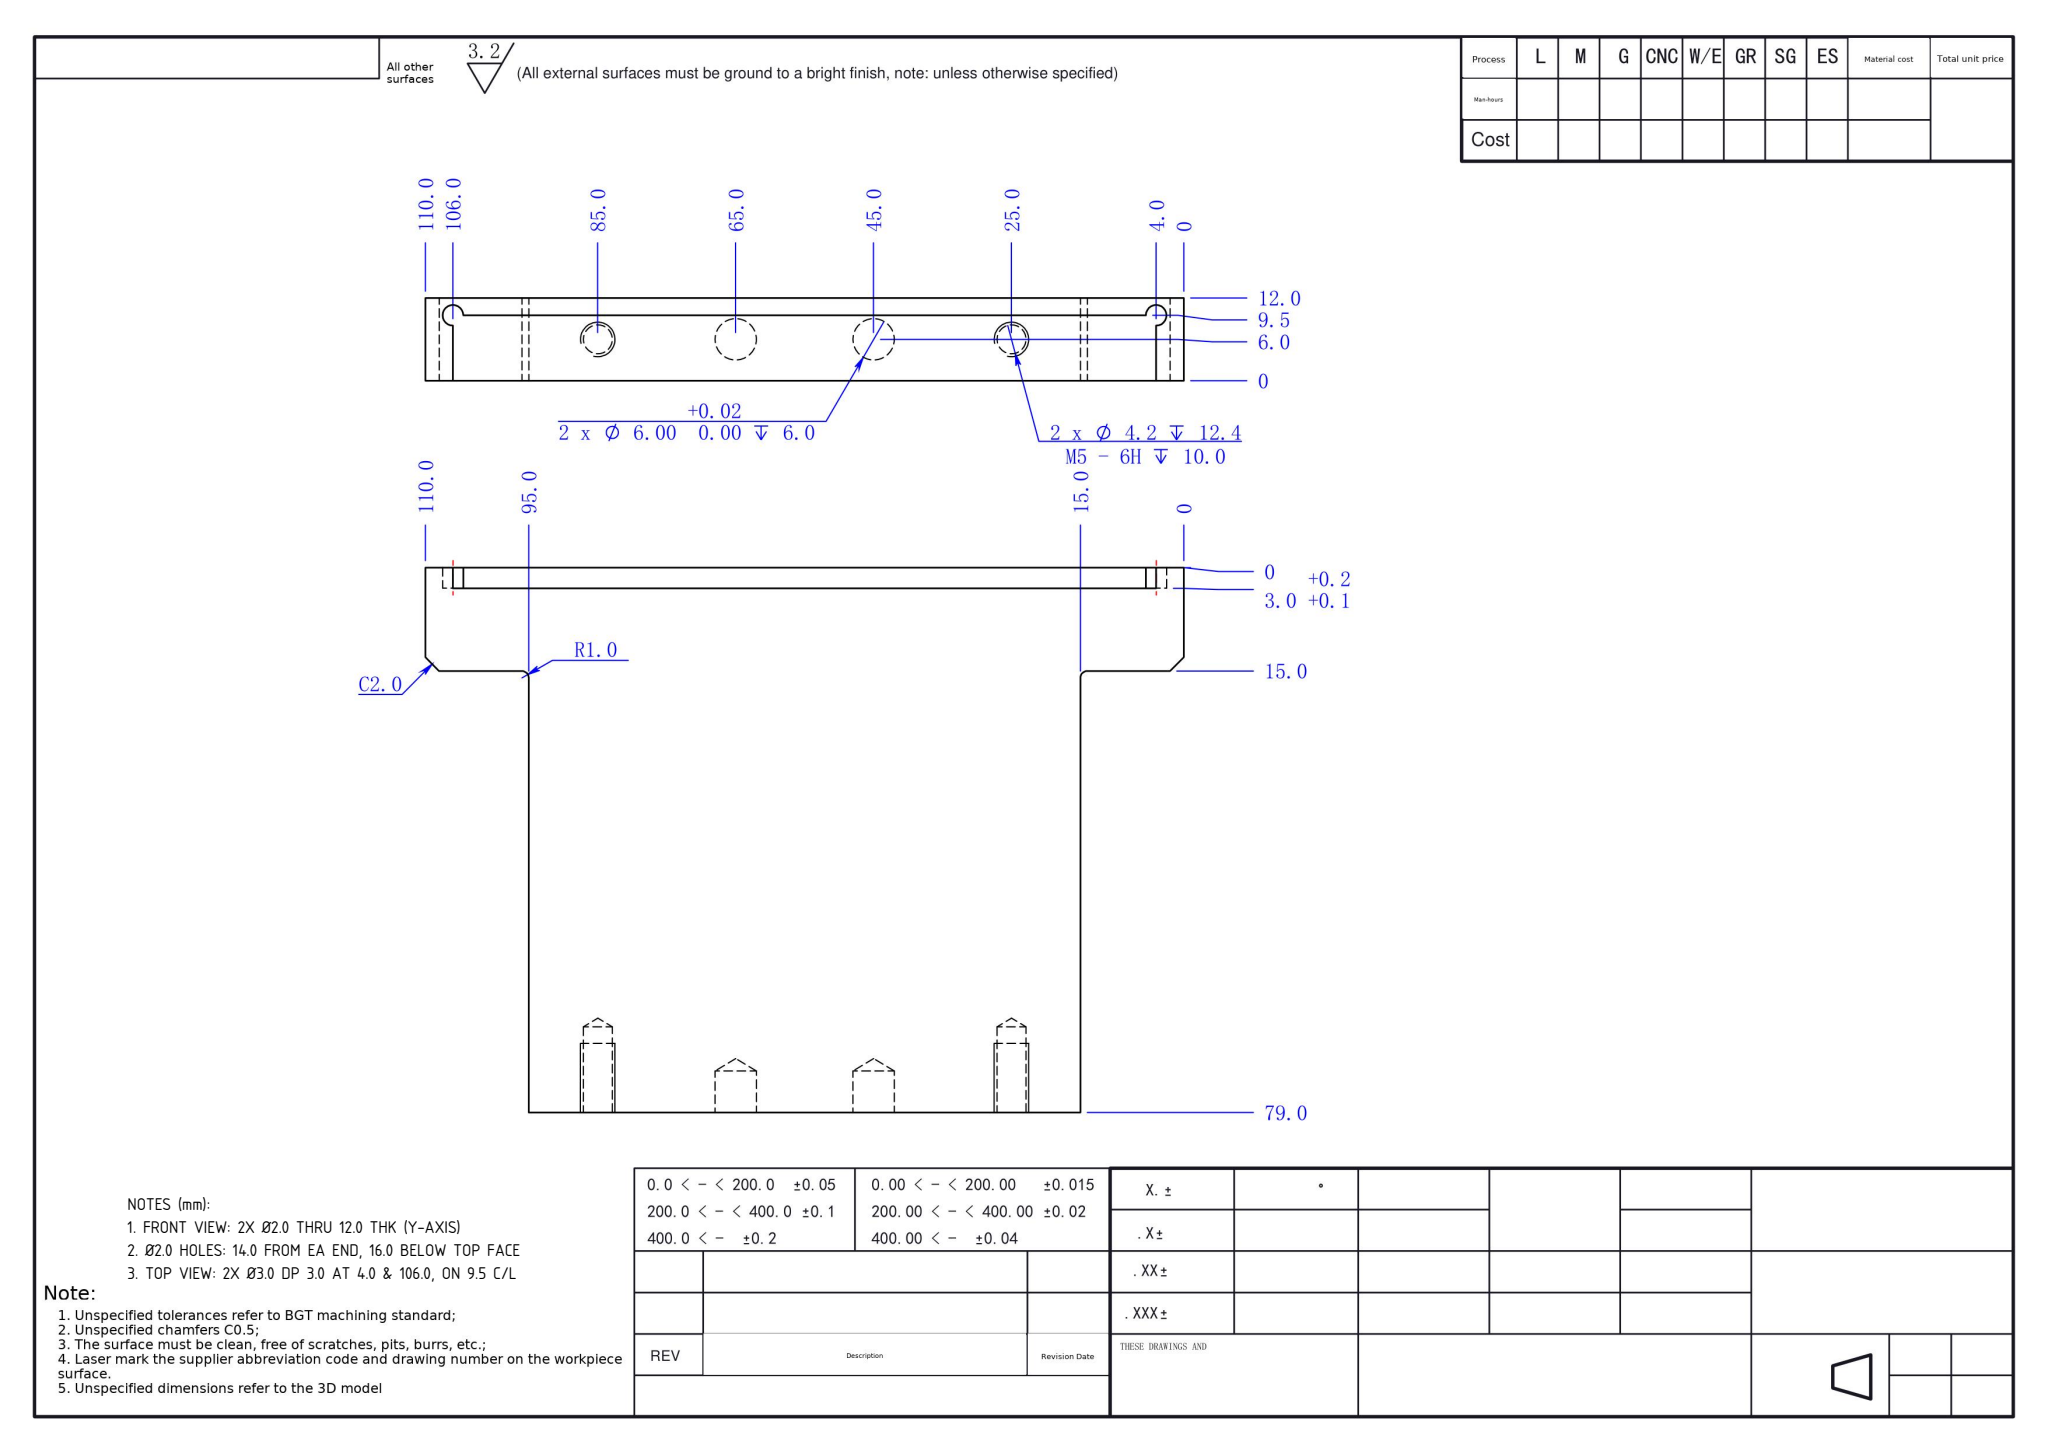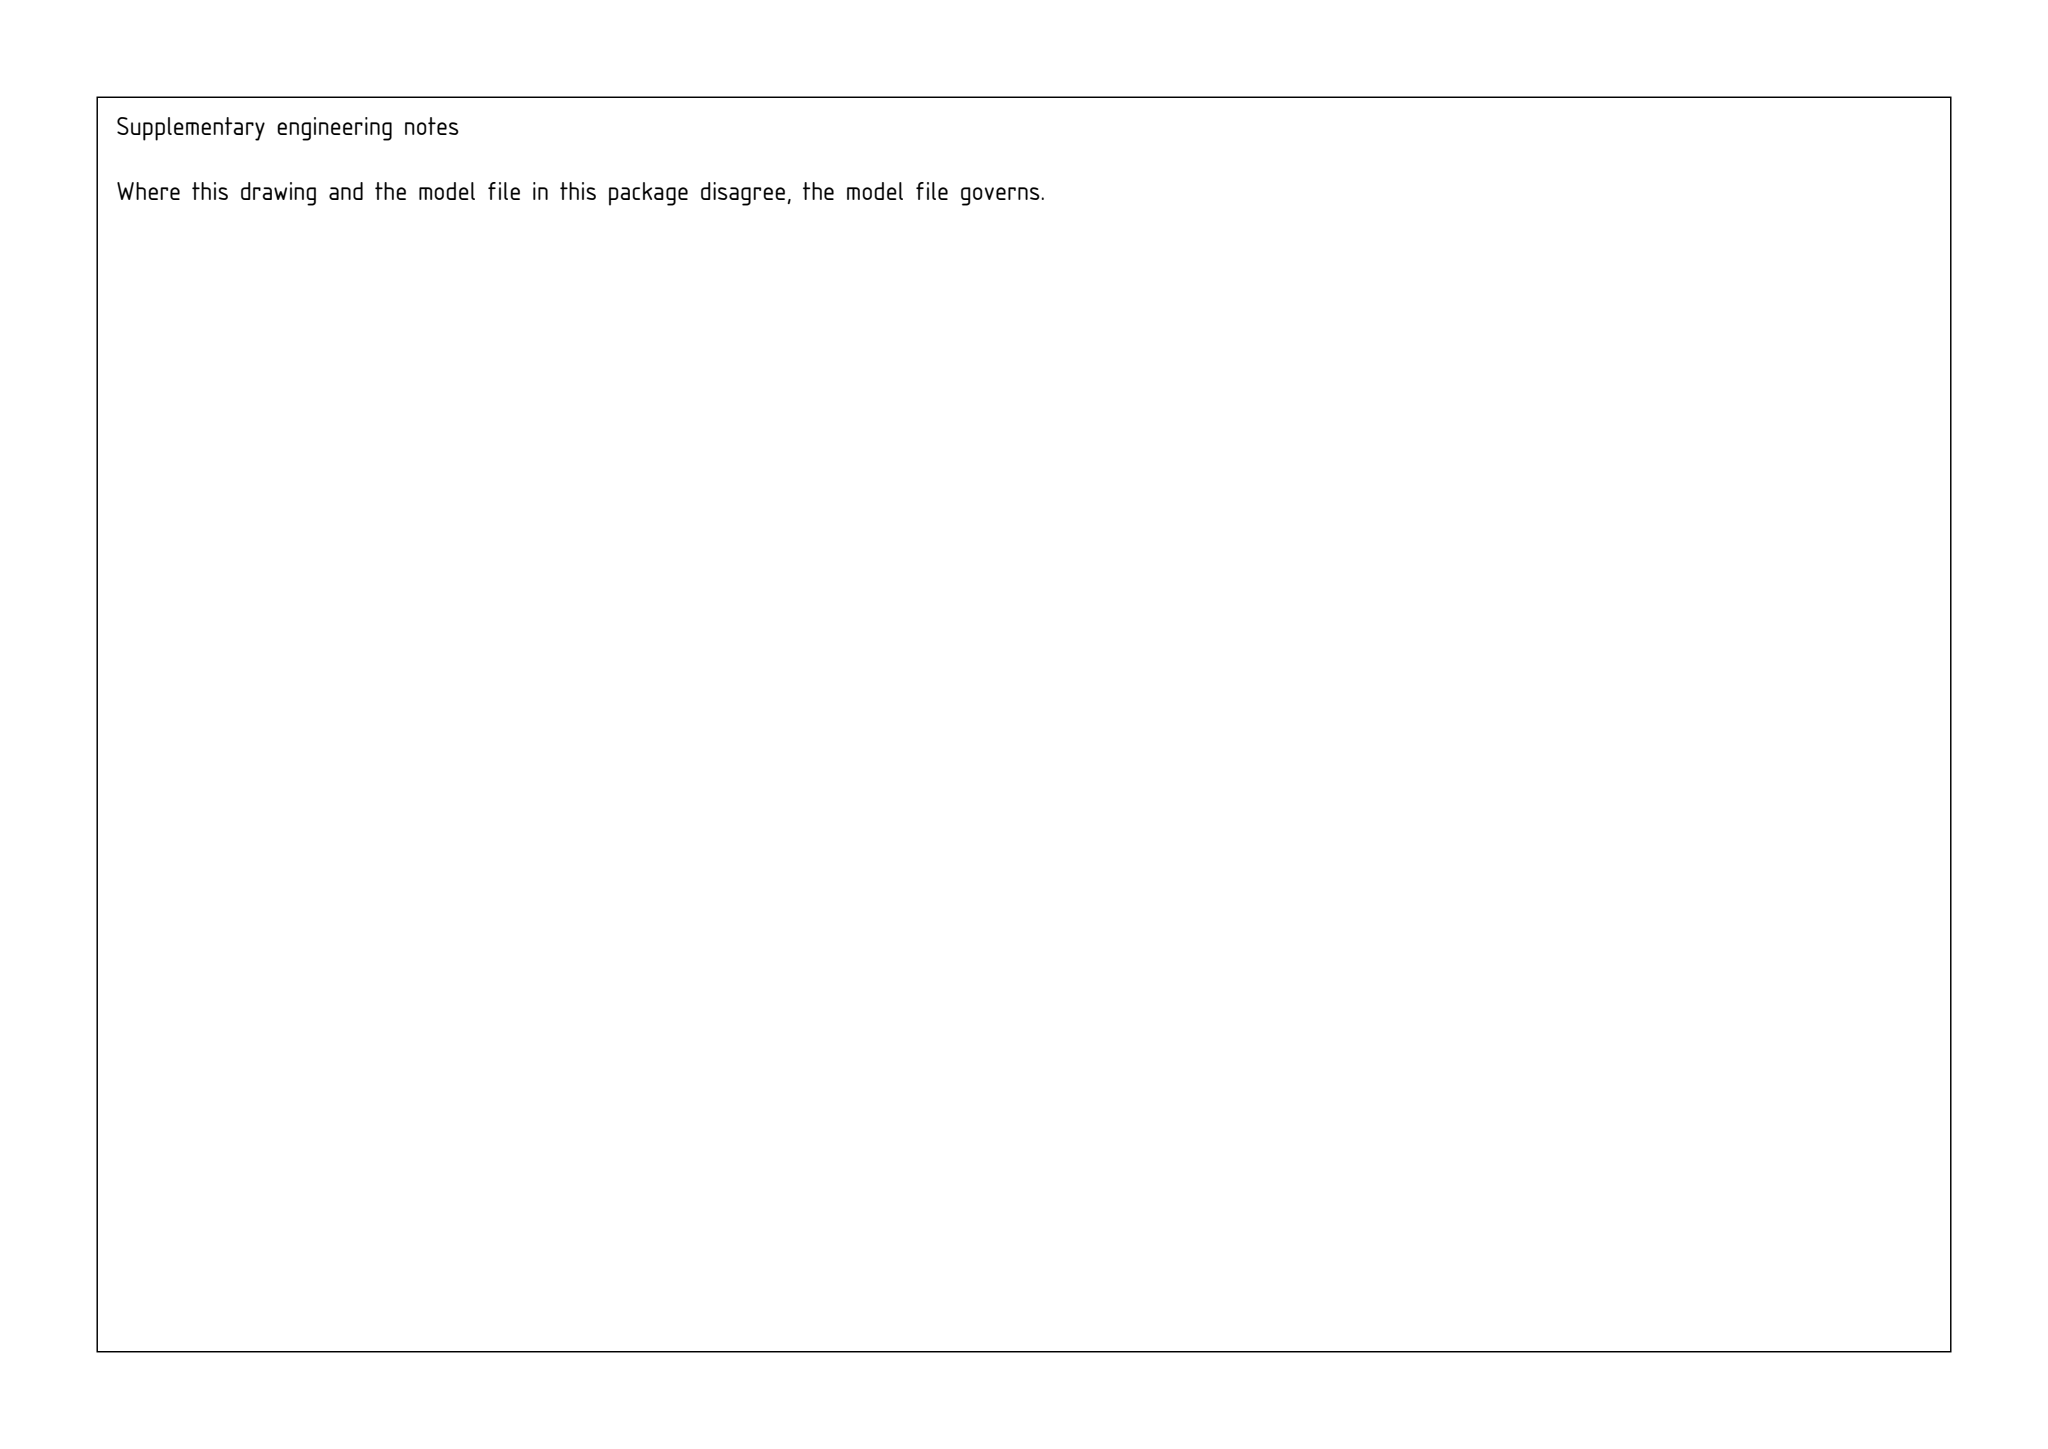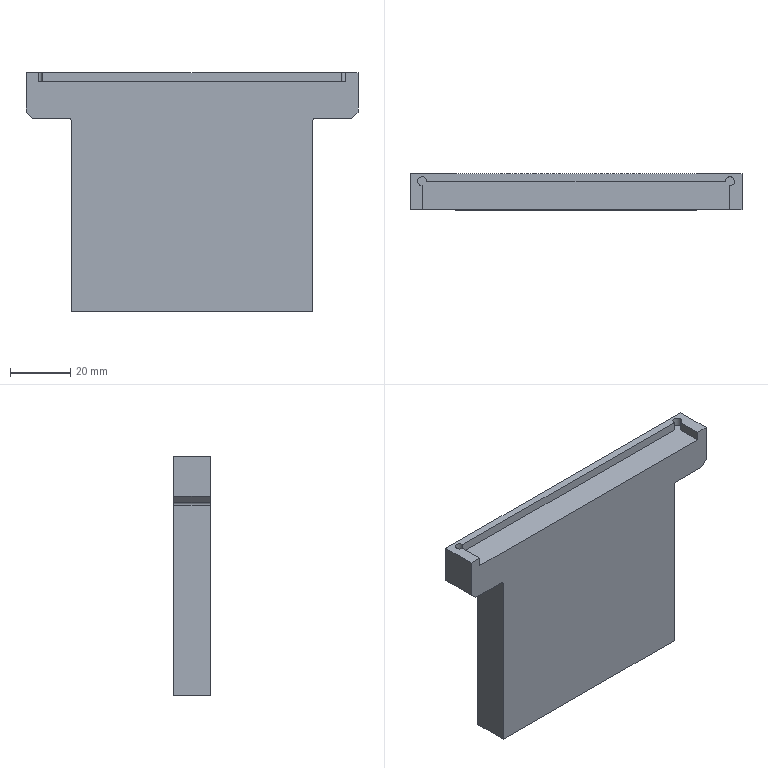Part | SolidWorks | mm | 1 solid | 37 faces | box 110 x 12 x 79 mm | volume 77530 mm3 | plane 16 | cylinder 13 | cone 8 | commonest cylinder face diameters 6 x4 4.2 x4 3 x3 2 x2
Drawing notes:
FRONT VIEW: 2X Ø2.0 THRU 12.0 THK (Y-AXIS) | from the solid: cylinders dia 2.0 axis y at (14,-,63) and (96,-,63), length 12.0 = full y thickness (y planes 0 and 12.0)
Ø2.0 HOLES: 14.0 FROM EA END, 16.0 BELOW TOP FACE | from the solid: hole axes at x=14.0 and x=96.0 of 110.0 overall; z=63.0 with top face z=79.0 -> 79.0-63.0=16.0
TOP VIEW: 2X Ø3.0 DP 3.0 AT 4.0 & 106.0, ON 9.5 C/L | from the solid: cylinders dia 3.0 axis z at (4.0,9.5) and (106.0,9.5), length 3.0
build123d program:
from build123d import *

# Parameters (mm, degrees)
SKETCH1_W                     = 120
SKETCH1_H                     = 20
BOSS_EXTRUDE1_DEPTH           = 9
SKETCH2_W                     = 116
SKETCH2_H                     = 18
CUT_EXTRUDE1_DEPTH            = 3
MOVE_FACE1_BY                 = 5
MOVE_FACE1_2_BY               = 5
MOVE_FACE2_BY                 = 5
MOVE_FACE2_2_BY               = 5
MOVE_FACE3_BY                 = 5
MOVE_FACE4_BY                 = 2
MOVE_FACE5_BY                 = 2
MOVE_FACE5_2_BY               = 2
SKETCH3_R                     = 1.5
CUT_EXTRUDE2_DEPTH            = 3
SKETCH6_W                     = 110
SKETCH6_H                     = 15
BOSS_EXTRUDE2_DEPTH           = 70
SKETCH7_W                     = 15
SKETCH7_H                     = 64
CUT_EXTRUDE3_DEPTH            = 148.078
FILLET1_R                     = 1
CHAMFER1_SIZE                 = 2
M5_TAPPED_HOLE1_D             = 4.2
M5_TAPPED_HOLE1_DEPTH         = 12.4
M5_TAPPED_HOLE1_TIP           = 1.262
SIZE_MM_DOWEL_PIN_HOLE1_D     = 6
SIZE_MM_DOWEL_PIN_HOLE1_DEPTH = 6
SIZE_MM_DOWEL_PIN_HOLE1_TIP   = 1.803
SKETCH12_W                    = 110
SKETCH12_H                    = 1.5
CUT_EXTRUDE4_DEPTH            = 152.618


with BuildPart() as part:
    # Sketch1 → Boss-Extrude1 (new body)
    with BuildSketch(Plane.XY):
        with Locations((-73.48, 5.49)):
            Rectangle(SKETCH1_W, SKETCH1_H)
    extrude(amount=BOSS_EXTRUDE1_DEPTH)

    # Sketch2 → Cut-Extrude1 (cut)
    with BuildSketch(Plane.XY.offset(9)):
        with Locations((-73.48, 4.49)):
            Rectangle(SKETCH2_W, SKETCH2_H)
    extrude(amount=-CUT_EXTRUDE1_DEPTH, mode=Mode.SUBTRACT)

    # Move Face1: a face moved outward by 5.0
    extrude(part.faces().sort_by_distance((-15.48, 4.49, 7.5))[0], amount=MOVE_FACE1_BY, dir=(-1, 0, 0))

    # Move Face1 2: a face moved outward by 5.0
    extrude(part.faces().sort_by_distance((-131.48, 4.49, 7.5))[0], amount=MOVE_FACE1_2_BY, dir=(1, 0, 0))

    # Move Face2: a face moved inward by 5.0
    extrude(part.faces().sort_by_distance((-13.48, 5.49, 4.5))[0], amount=MOVE_FACE2_BY, dir=(-1, 0, 0), mode=Mode.SUBTRACT)

    # Move Face2 2: a face moved inward by 5.0
    extrude(part.faces().sort_by_distance((-133.48, 5.49, 4.5))[0], amount=MOVE_FACE2_2_BY, dir=(1, 0, 0), mode=Mode.SUBTRACT)

    # Move Face3: a face moved inward by 5.0
    extrude(part.faces().sort_by_distance((-73.48, -4.51, 3.08))[0], amount=MOVE_FACE3_BY, dir=(0, 1, 0), mode=Mode.SUBTRACT)

    # Move Face4: a face moved outward by 2.0
    extrude(part.faces().sort_by_distance((-73.48, 13.49, 7.5))[0], amount=MOVE_FACE4_BY, dir=(0, -1, 0))

    # Move Face5: a face moved outward by 2.0
    extrude(part.faces().sort_by_distance((-126.48, 5.99, 7.5))[0], amount=MOVE_FACE5_BY, dir=(1, 0, 0))

    # Move Face5 2: a face moved outward by 2.0
    extrude(part.faces().sort_by_distance((-20.48, 5.99, 7.5))[0], amount=MOVE_FACE5_2_BY, dir=(-1, 0, 0))

    # Sketch3 → Cut-Extrude2 (cut)
    with BuildSketch(Plane.XY.offset(9)):
        with Locations((-124.48, 11.49)):
            Circle(SKETCH3_R)
        with Locations((-22.48, 11.49)):
            Circle(SKETCH3_R)
    extrude(amount=-CUT_EXTRUDE2_DEPTH, mode=Mode.SUBTRACT)

    # Sketch6 → Boss-Extrude2 (add)
    with BuildSketch(Plane(origin=(0, 0, 0), x_dir=(-1, 0, 0), z_dir=(0, 0, -1))):
        with Locations((73.48, 7.99)):
            Rectangle(SKETCH6_W, SKETCH6_H)
    extrude(amount=BOSS_EXTRUDE2_DEPTH)

    # Sketch7 → Cut-Extrude3 (cut, through all)
    with BuildSketch(Plane.XZ.offset(-0.4902)):
        with Locations((-120.98, -38)):
            Rectangle(SKETCH7_W, SKETCH7_H)
        with Locations((-25.98, -38)):
            Rectangle(SKETCH7_W, SKETCH7_H)
    extrude(amount=-CUT_EXTRUDE3_DEPTH, mode=Mode.SUBTRACT)

    # Fillet1
    fillet1_edges = [part.edges().sort_by_distance(p)[0] for p in [
        (-113.48, 7.99, -6),
        (-33.48, 7.99, -6),
    ]]
    fillet(fillet1_edges, radius=FILLET1_R)

    # Chamfer1
    chamfer1_edges = [part.edges().sort_by_distance(p)[0] for p in [
        (-128.48, 7.99, -6),
        (-18.48, 7.99, -6),
    ]]
    chamfer(chamfer1_edges, length=CHAMFER1_SIZE)

    # M5 Tapped Hole1
    with Locations(Plane(origin=(0, 0, -70), x_dir=(-1, 0, 0), z_dir=(0, 0, -1))):
        with Locations((43.48, 7.99), (103.48, 7.99)):
            Hole(M5_TAPPED_HOLE1_D / 2, depth=M5_TAPPED_HOLE1_DEPTH)
            with Locations((0, 0, -(M5_TAPPED_HOLE1_DEPTH + M5_TAPPED_HOLE1_TIP / 2))):  # 118° drill point
                Cone(0, M5_TAPPED_HOLE1_D / 2, M5_TAPPED_HOLE1_TIP, mode=Mode.SUBTRACT)

    # Size mm Dowel Pin Hole1
    with Locations(Plane(origin=(0, 0, -70), x_dir=(-1, 0, 0), z_dir=(0, 0, -1))):
        with Locations((63.48, 7.99), (83.48, 7.99)):
            Hole(SIZE_MM_DOWEL_PIN_HOLE1_D / 2, depth=SIZE_MM_DOWEL_PIN_HOLE1_DEPTH)
            with Locations((0, 0, -(SIZE_MM_DOWEL_PIN_HOLE1_DEPTH + SIZE_MM_DOWEL_PIN_HOLE1_TIP / 2))):  # 118° drill point
                Cone(0, SIZE_MM_DOWEL_PIN_HOLE1_D / 2, SIZE_MM_DOWEL_PIN_HOLE1_TIP, mode=Mode.SUBTRACT)

    # Sketch12 → Cut-Extrude4 (cut, through all)
    with BuildSketch(Plane(origin=(0, 0, -70), x_dir=(-1, 0, 0), z_dir=(0, 0, -1))):
        with Locations((73.48, 1.24)):
            Rectangle(SKETCH12_W, SKETCH12_H)
        with Locations((73.48, 14.74)):
            Rectangle(SKETCH12_W, SKETCH12_H)
    extrude(amount=-CUT_EXTRUDE4_DEPTH, mode=Mode.SUBTRACT)


solid = part.part